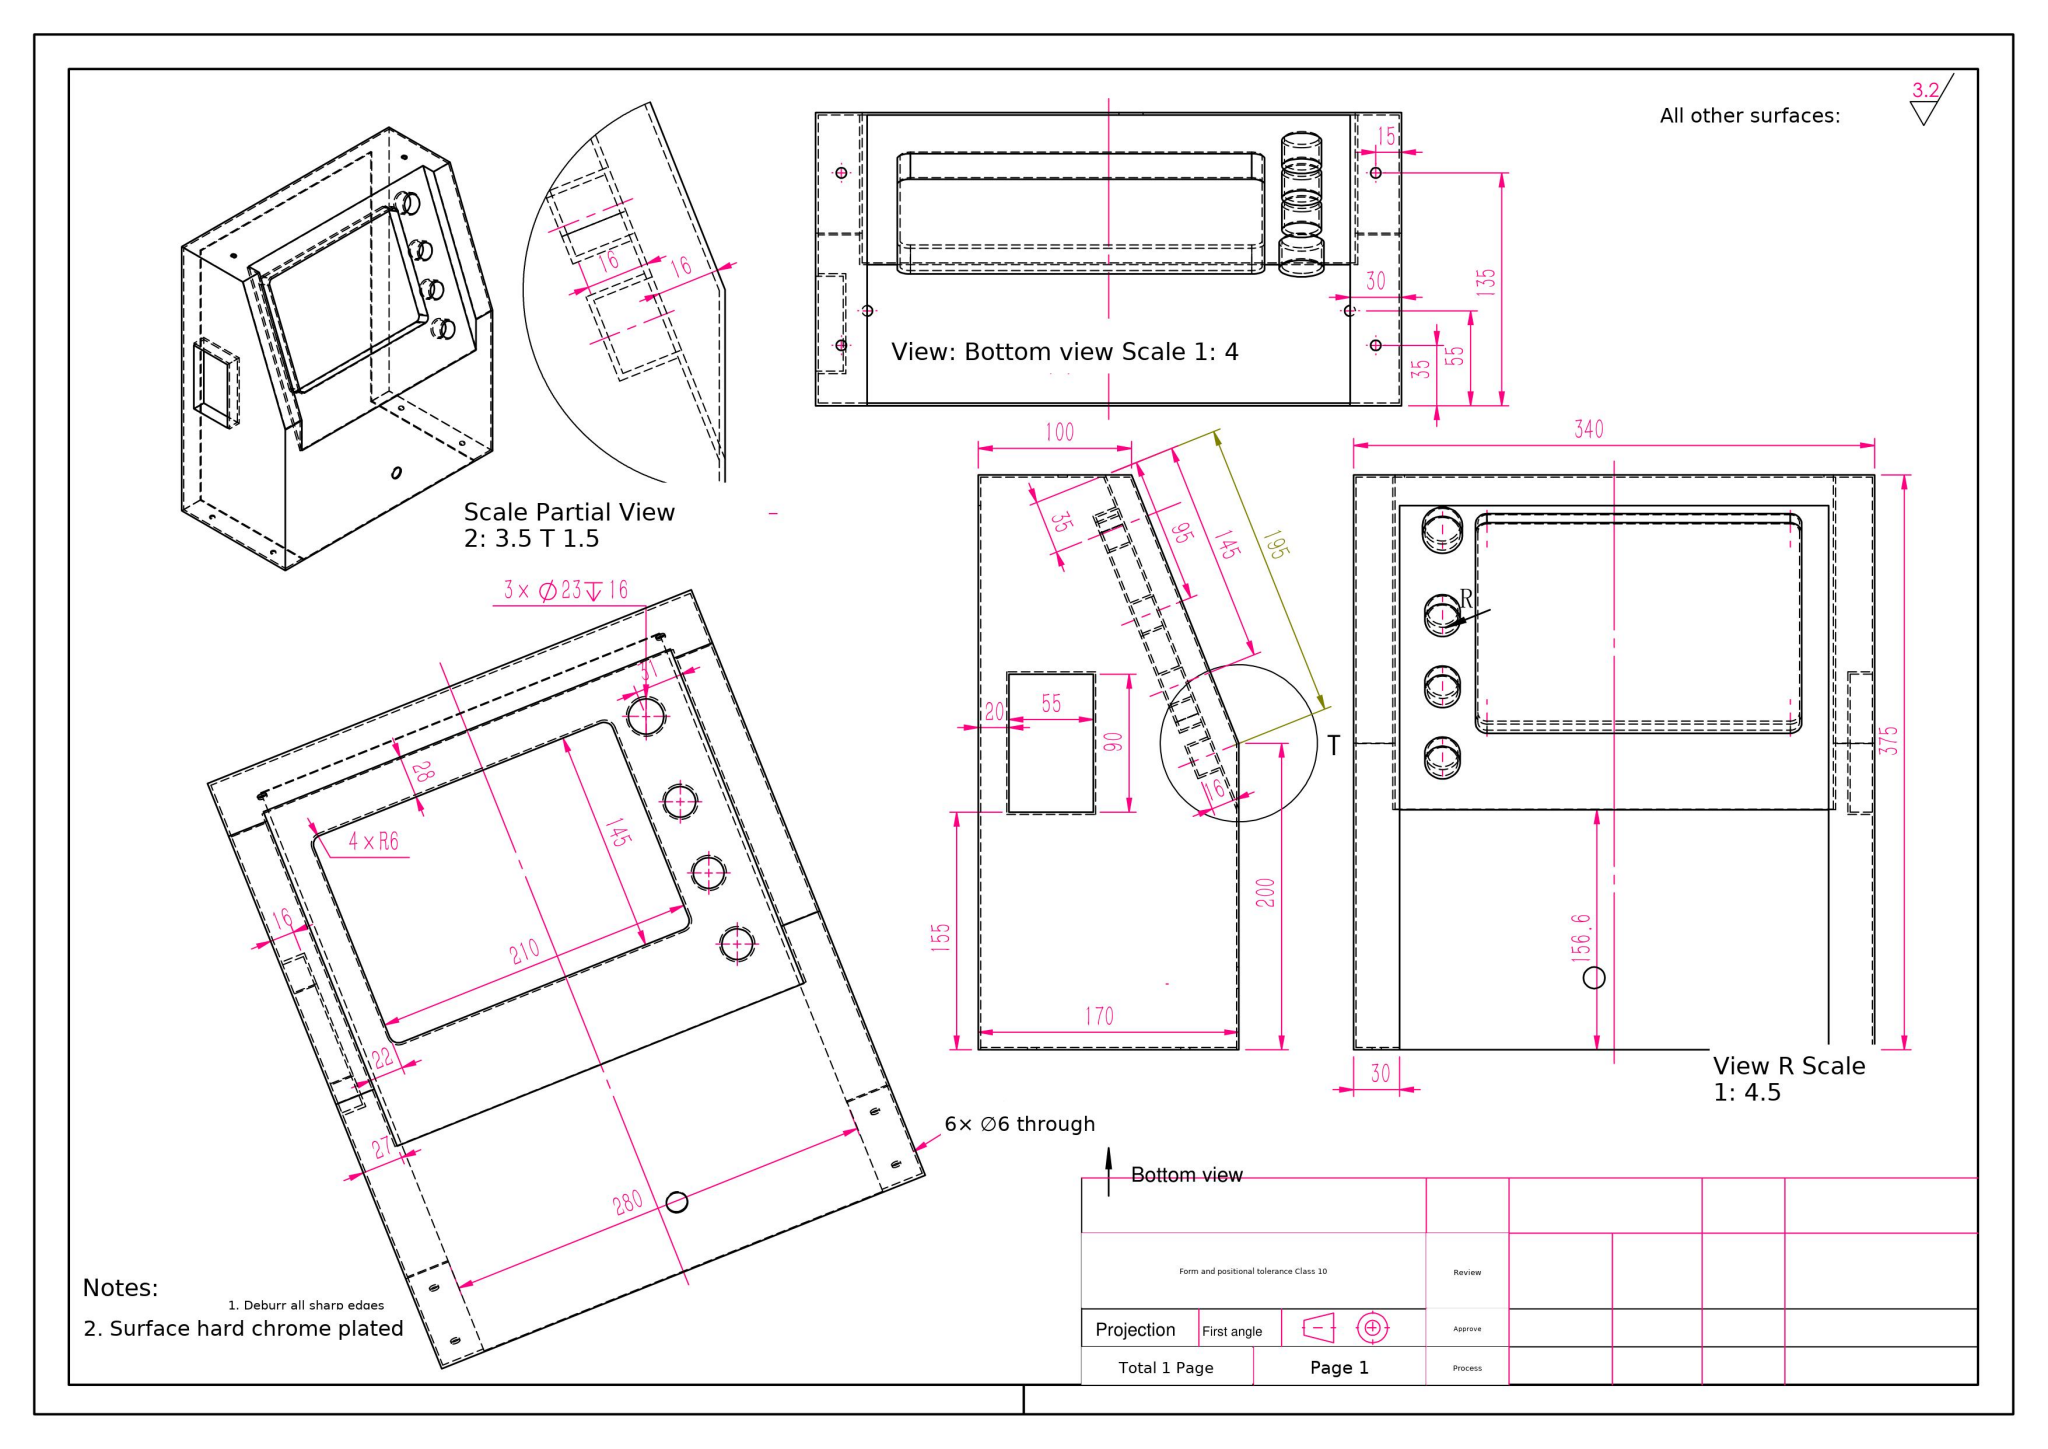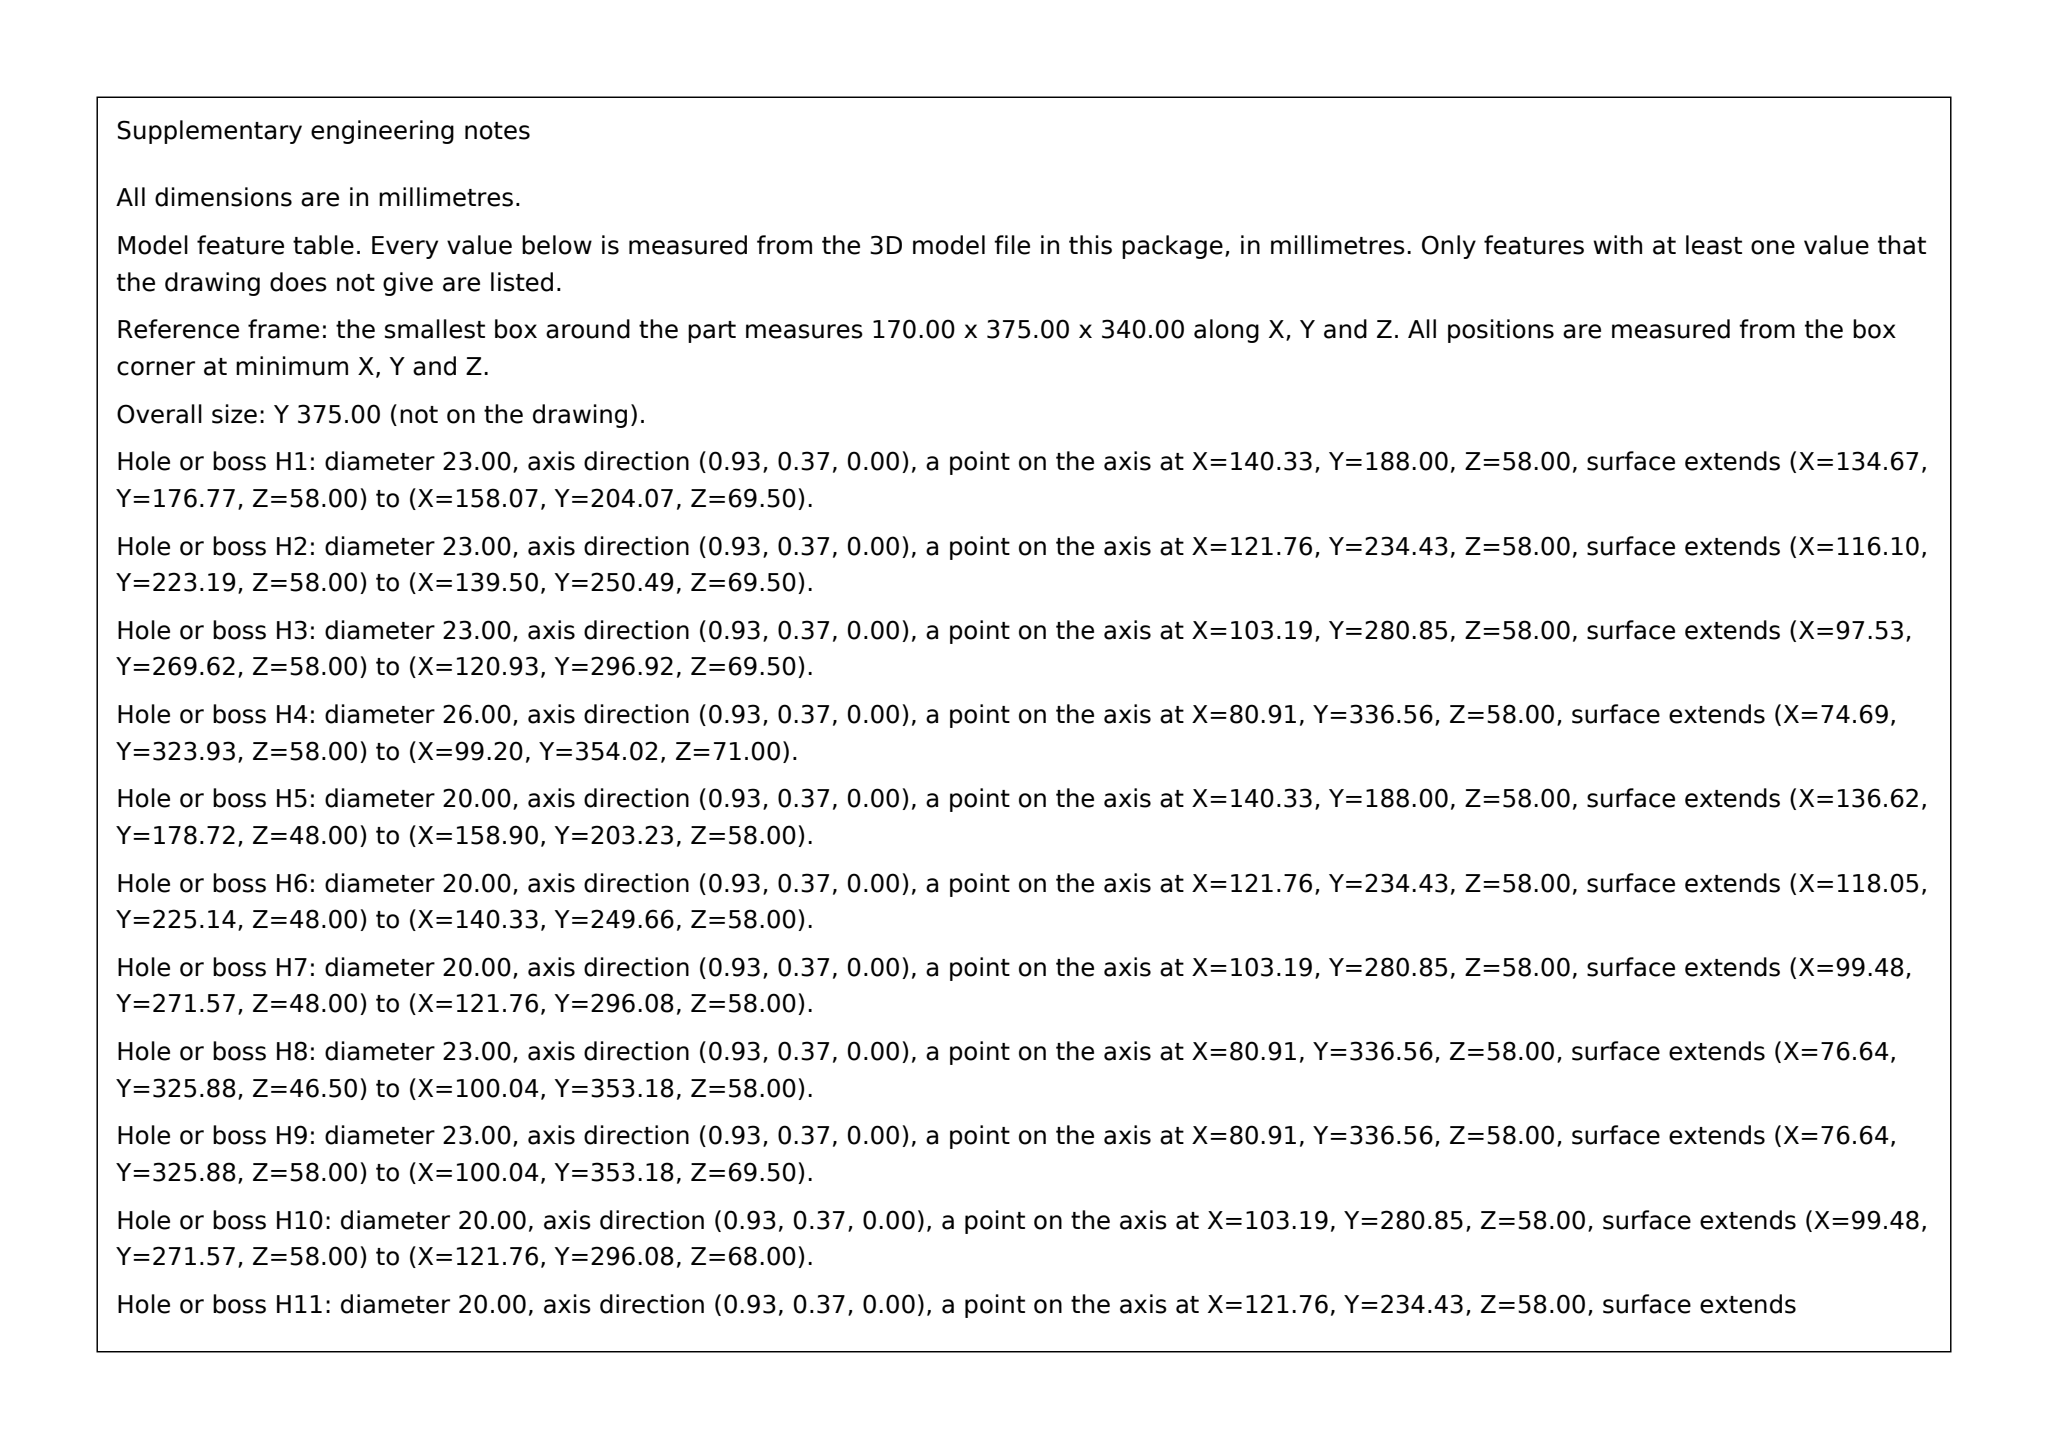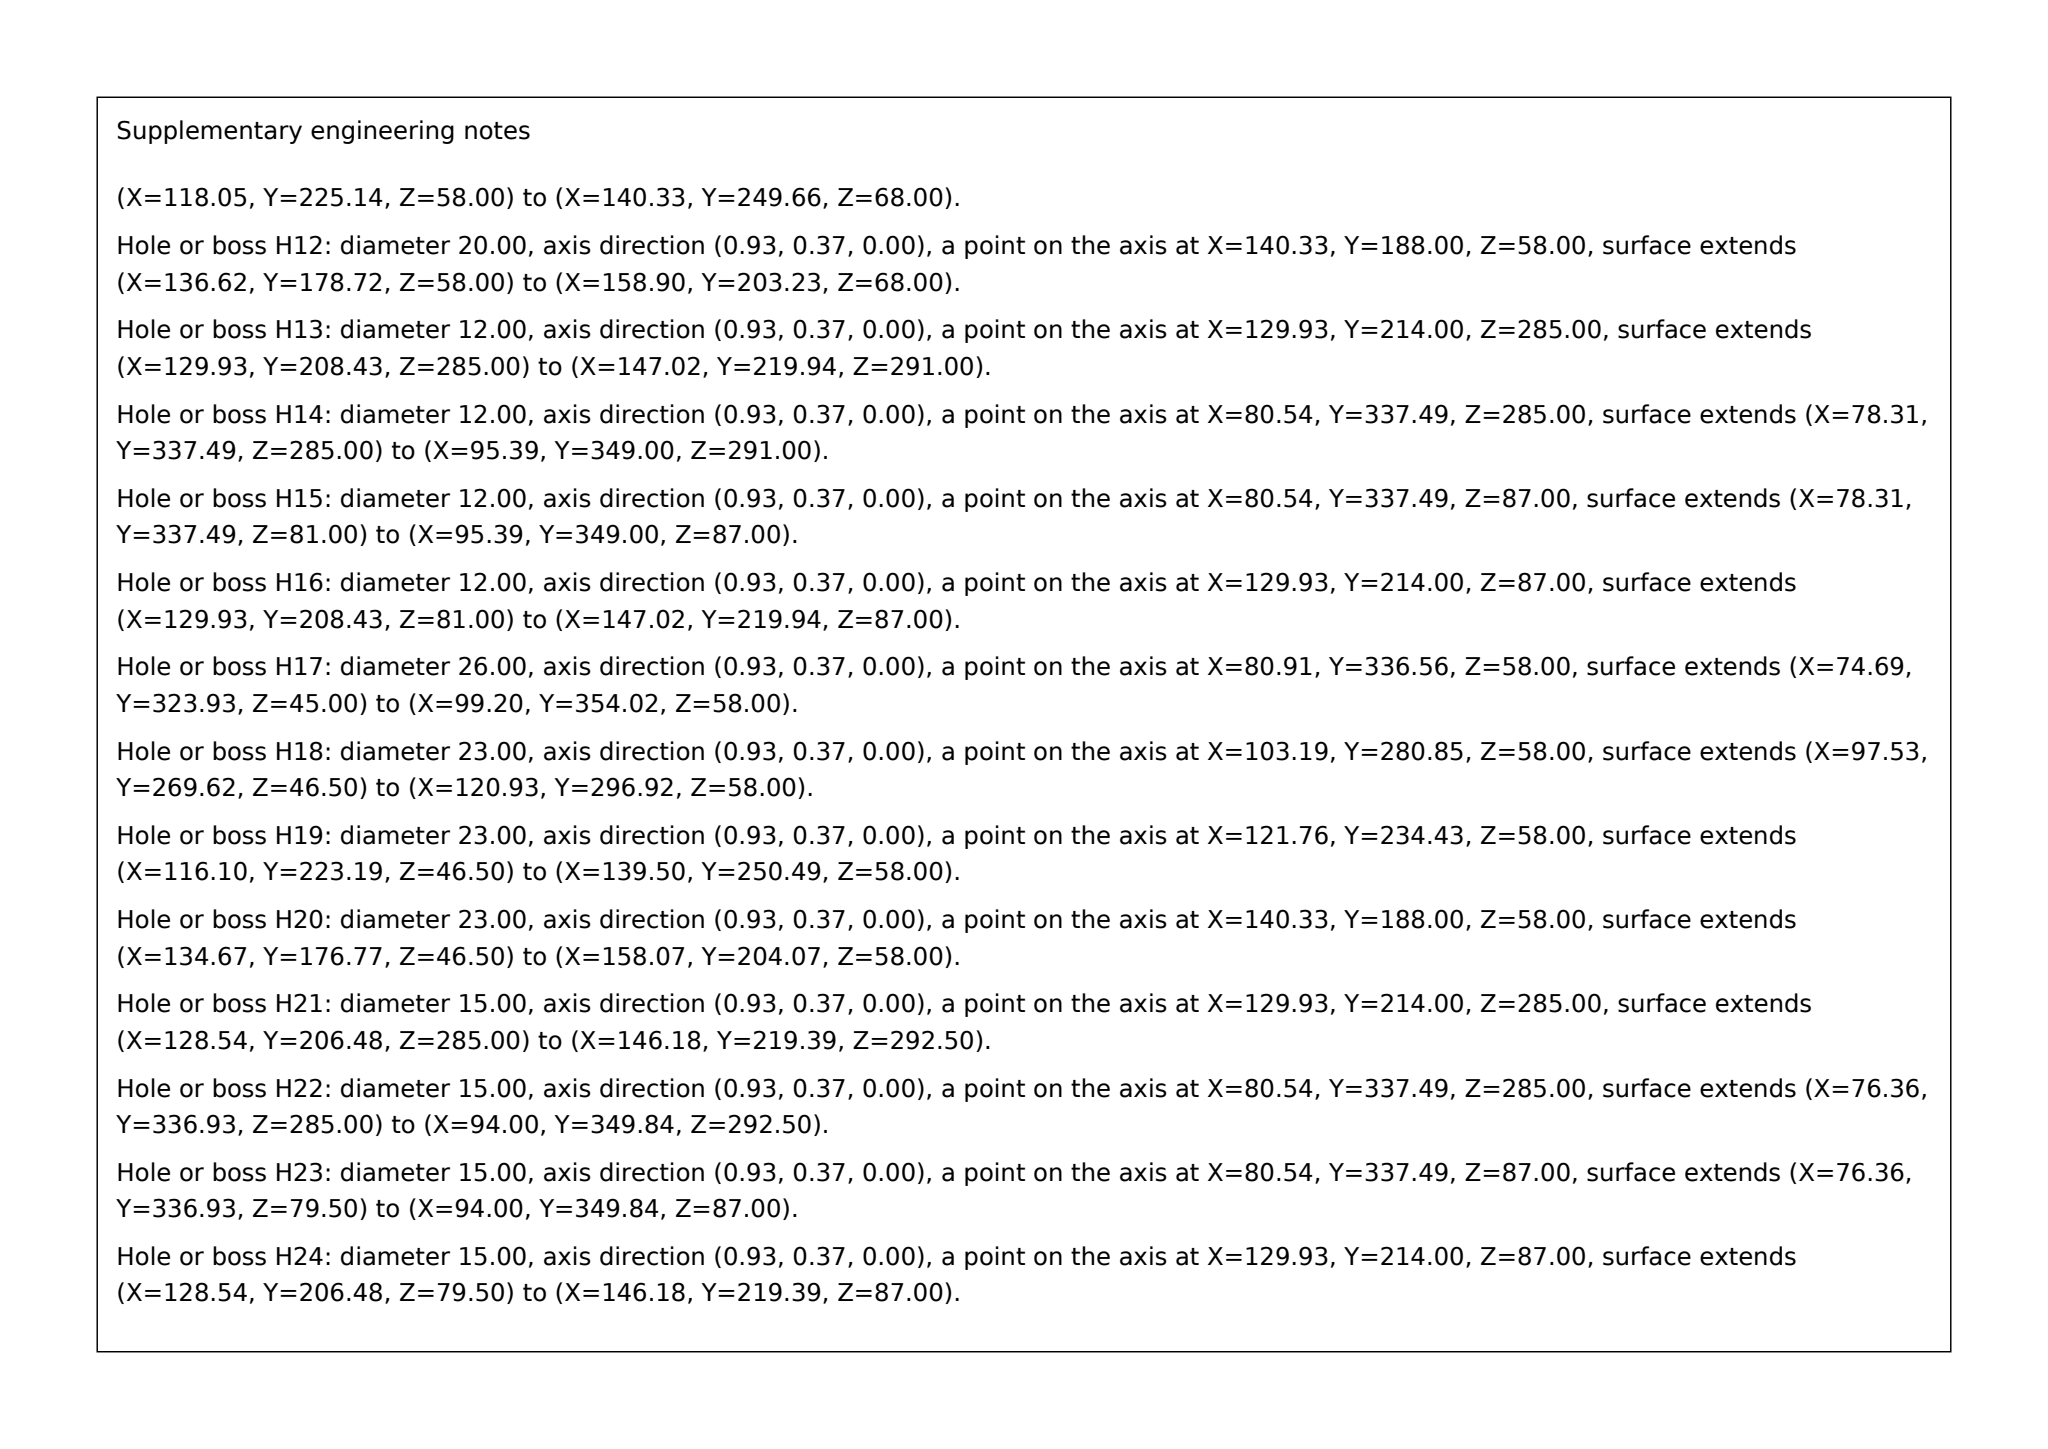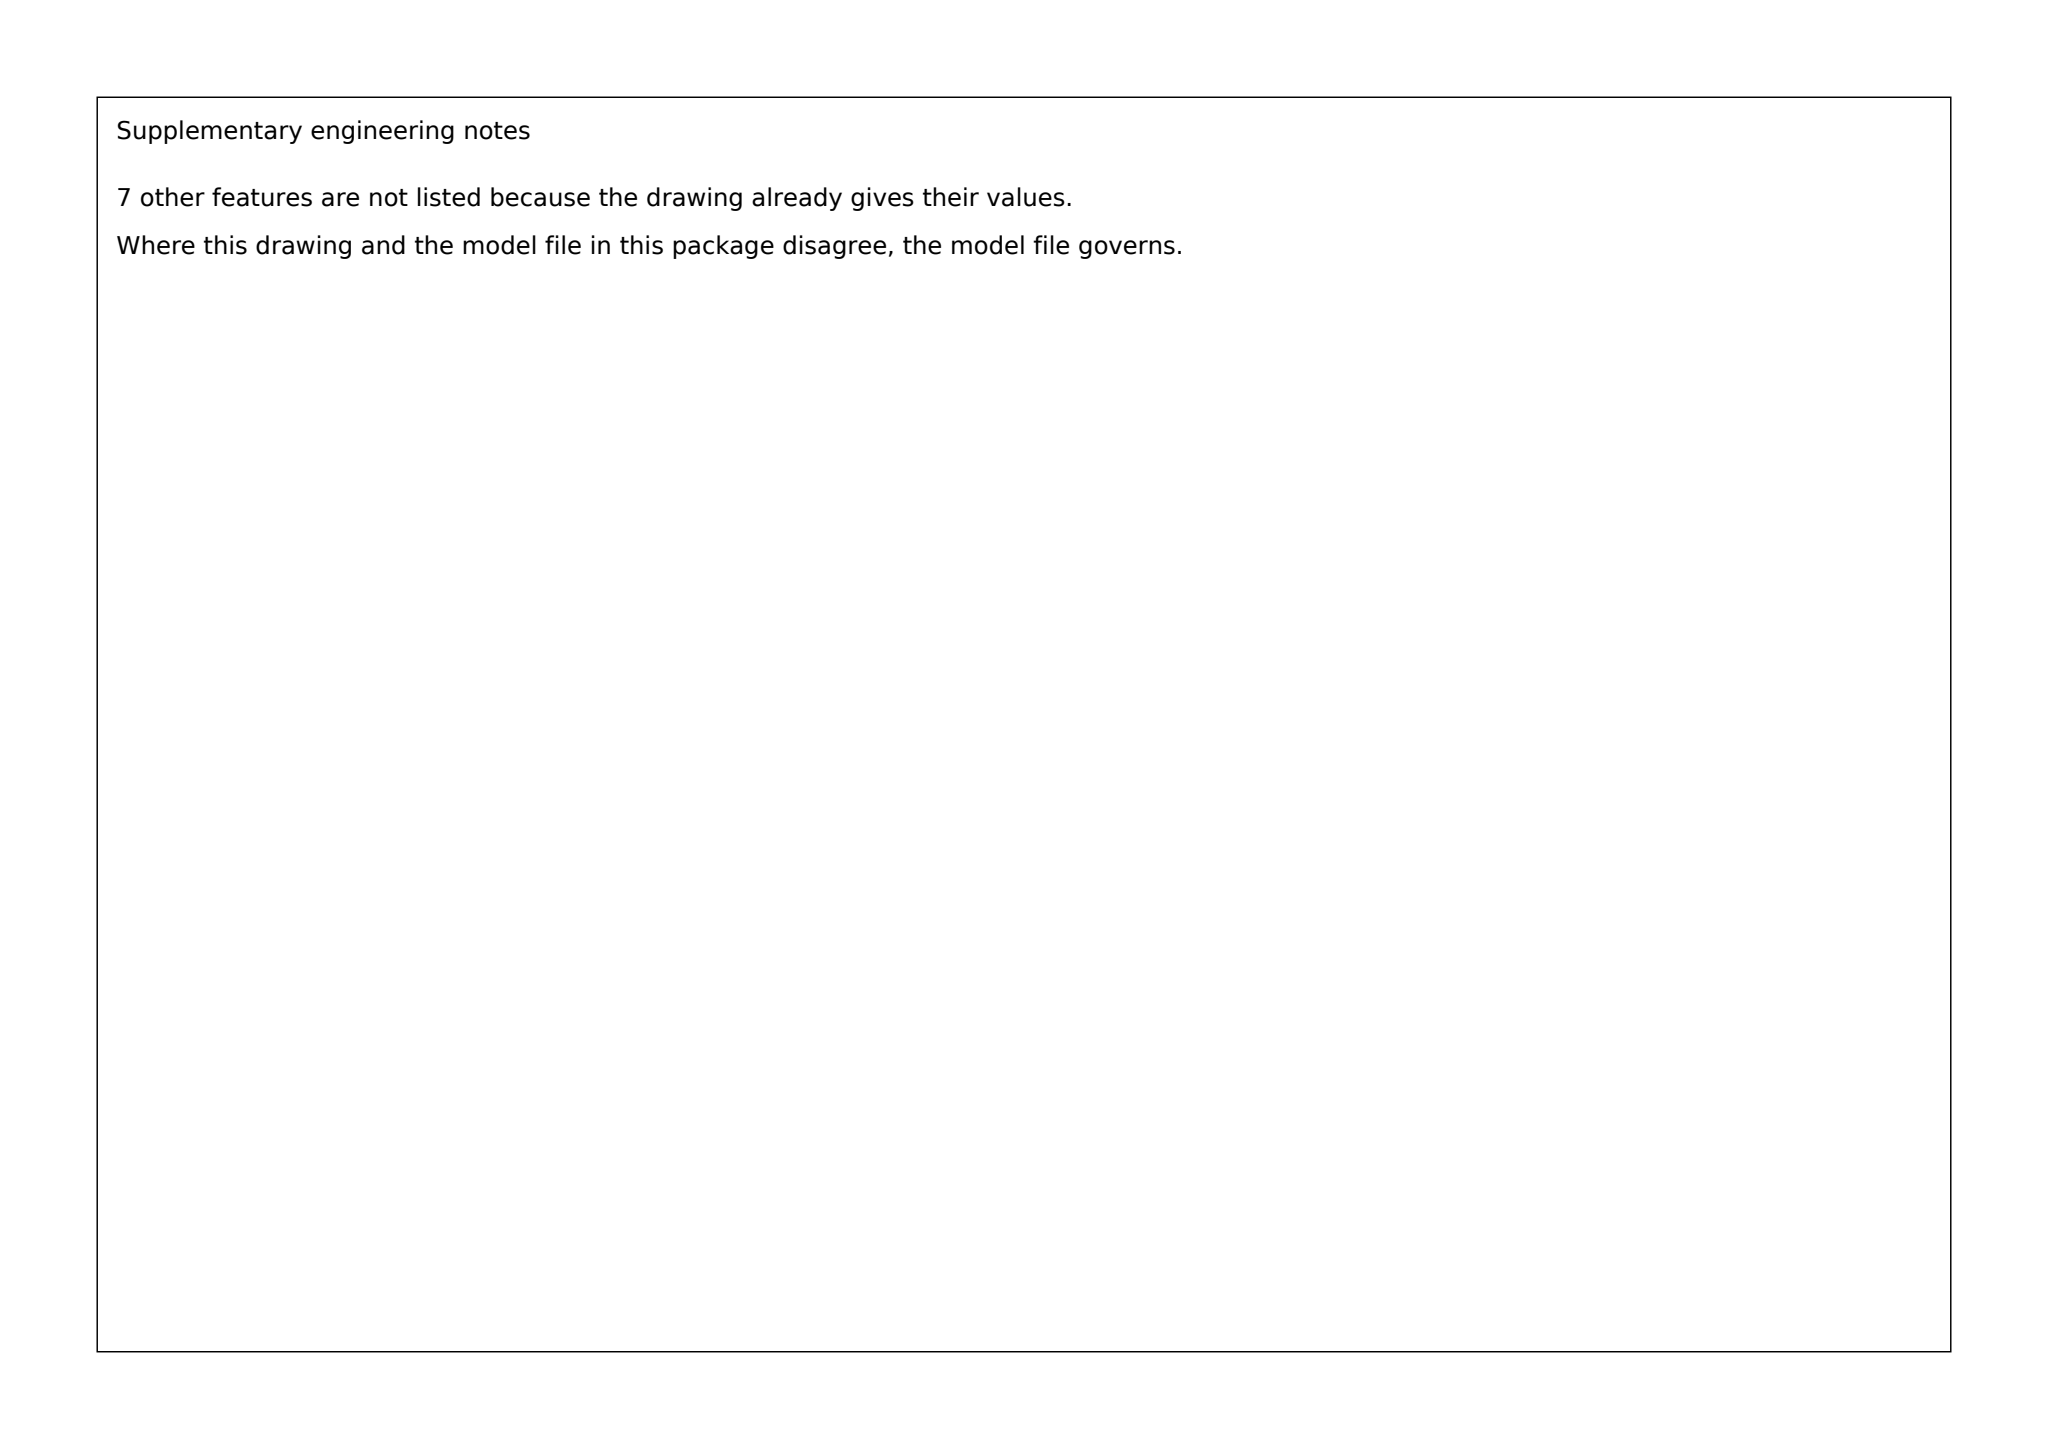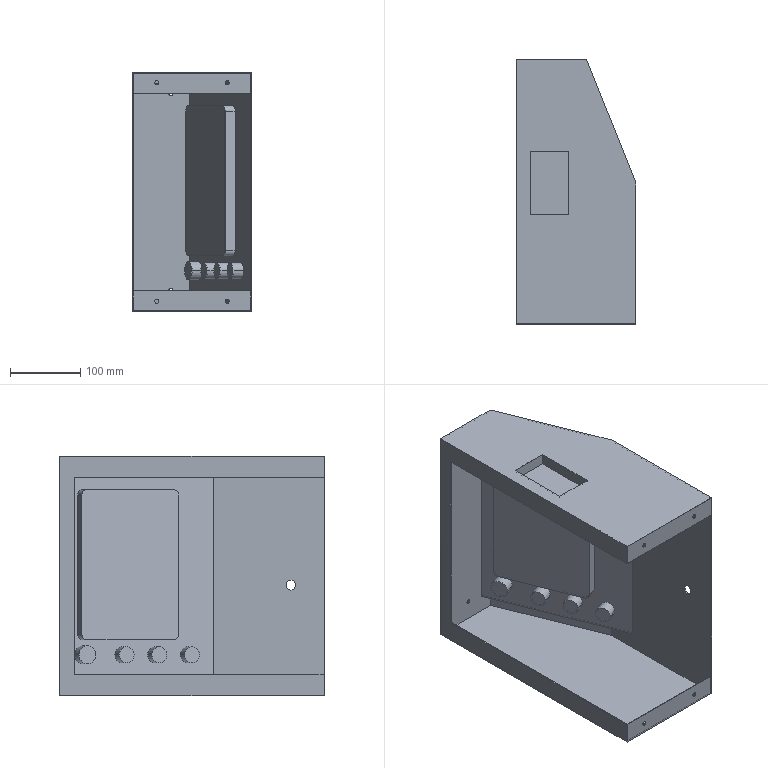Part | SolidWorks | mm | 1 solid | 93 faces | box 170 x 375 x 340 mm | volume 507424 mm3 | plane 55 | cylinder 38 | commonest cylinder face diameters 6 x8 23 x8 20 x6 6.2 x4 12 x4 15 x4 14 x2 26 x2